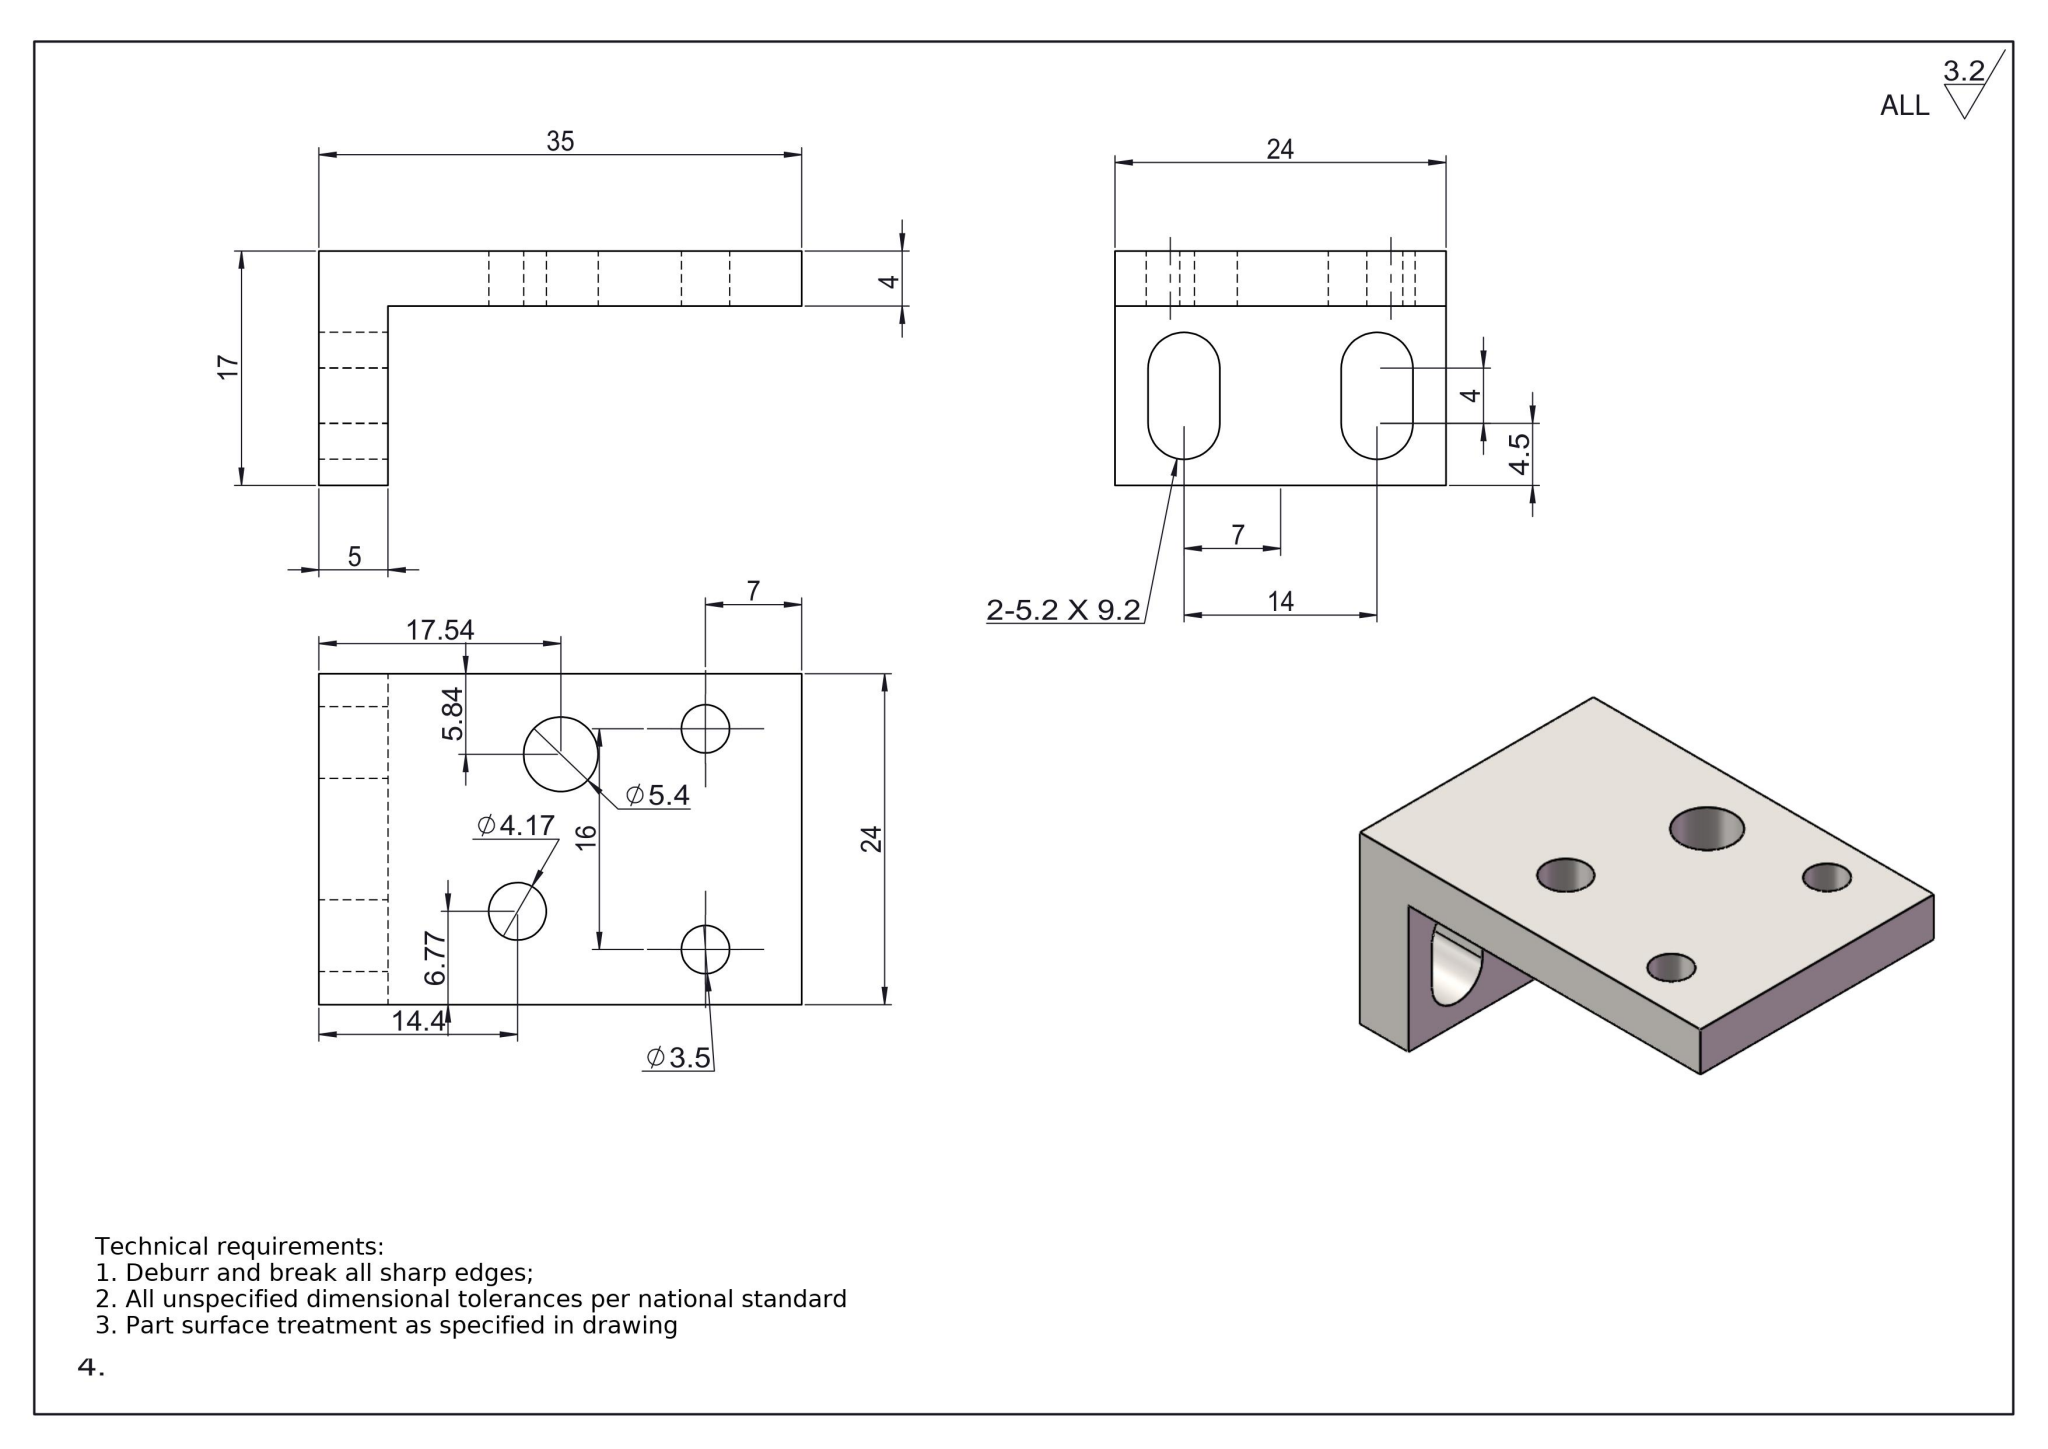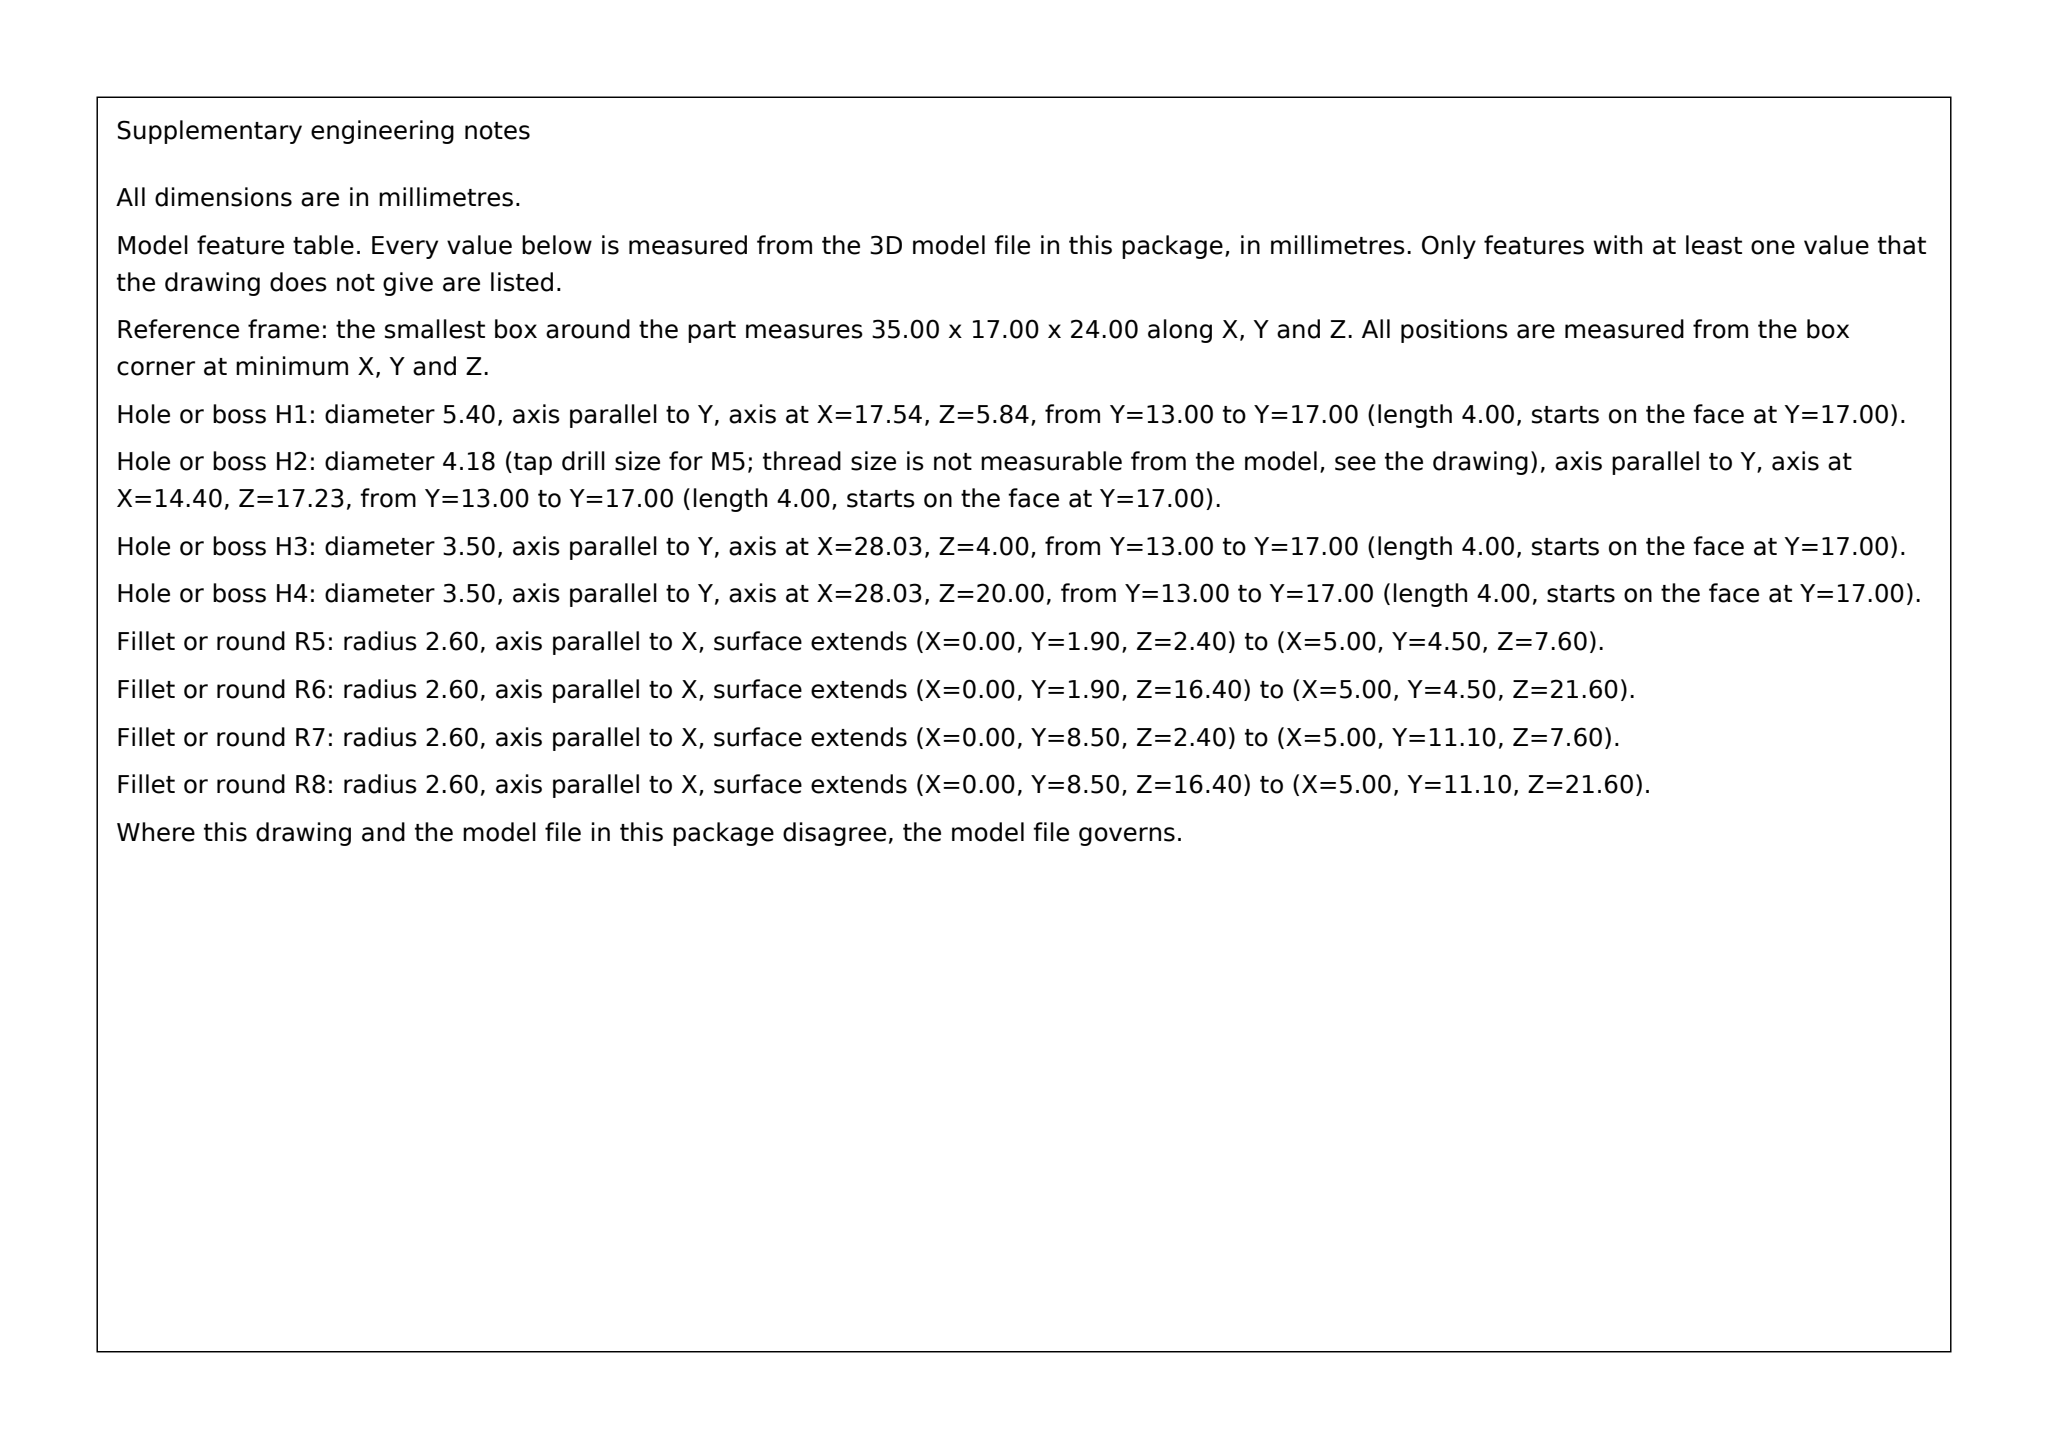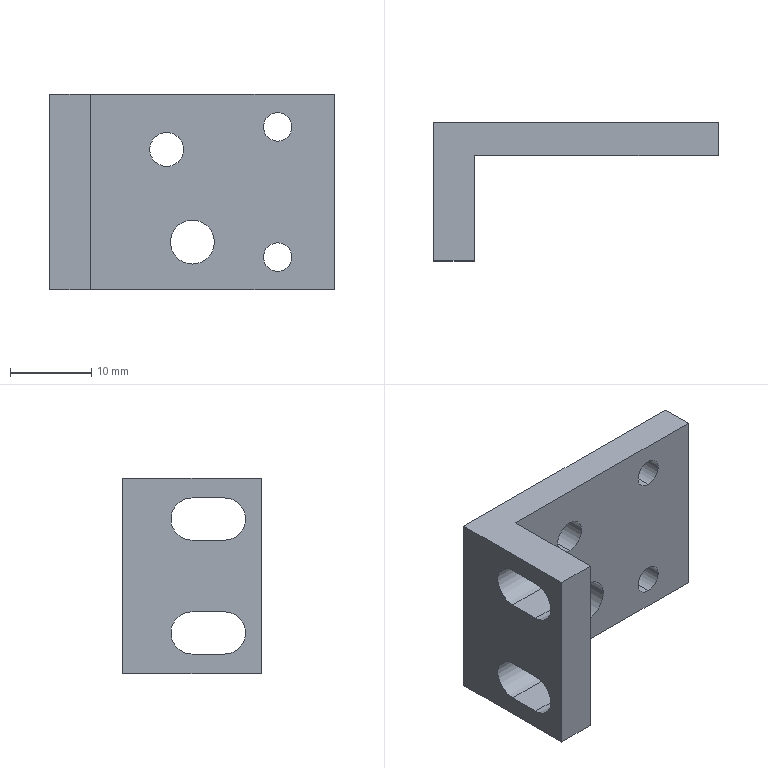Part | SolidWorks | mm | 1 solid | 24 faces | box 35 x 17 x 24 mm | volume 4276 mm3 | cylinder 12 | plane 12 | commonest cylinder face diameters 3.5 x4 5.2 x4 4.172 x2 5.404 x2
build123d program:
from build123d import *

# Parameters (mm, degrees)
BOSS_EXTRUDE1_DEPTH = 24
SKETCH2_R           = 1.75
CUT_EXTRUDE1_DEPTH  = 60.639
CUT_EXTRUDE2_DEPTH  = 46.946
SKETCH4_R           = 2.086
SKETCH4_R_2         = 2.702
CUT_EXTRUDE3_DEPTH  = 80


with BuildPart() as part:
    # Sketch1 → Boss-Extrude1 (new body)
    with BuildSketch(Plane.XY):
        Polygon((-53.027, -8.2), (-53.027, -25.2), (-48.027, -25.2), (-48.027, -12.2), (-18.027, -12.2), (-18.027, -8.2), align=None)
    extrude(amount=-BOSS_EXTRUDE1_DEPTH)

    # Sketch2 → Cut-Extrude1 (cut, through all)
    with BuildSketch(Plane.XZ.offset(12.2)):
        with Locations(Location((-25, -20, 0), (0, 0, 270))):
            Circle(SKETCH2_R)
        with Locations(Location((-25, -4, 0), (0, 0, 270))):
            Circle(SKETCH2_R)
    extrude(amount=-CUT_EXTRUDE1_DEPTH, mode=Mode.SUBTRACT)

    # Sketch3 → Cut-Extrude2 (cut, through all)
    with BuildSketch(Plane(origin=(-48.027, 0, 0), x_dir=(0, 0, -1), z_dir=(1, 0, 0))):
        with BuildLine():
            Line((7.6, -16.7), (7.6, -20.7))
            ThreePointArc((7.6, -20.7), (5, -23.3), (2.4, -20.7))
            Line((2.4, -20.7), (2.4, -16.7))
            ThreePointArc((2.4, -16.7), (5, -14.1), (7.6, -16.7))
        make_face()
        with BuildLine():
            Line((21.6, -16.7), (21.6, -20.7))
            ThreePointArc((21.6, -20.7), (19, -23.3), (16.4, -20.7))
            Line((16.4, -20.7), (16.4, -16.7))
            ThreePointArc((16.4, -16.7), (19, -14.1), (21.6, -16.7))
        make_face()
    extrude(amount=-CUT_EXTRUDE2_DEPTH, mode=Mode.SUBTRACT)

    # Sketch4 → Cut-Extrude3 (cut)
    with BuildSketch(Plane.XZ.offset(12.2)):
        with Locations(Location((-38.629, -6.772, 0), (0, 0, 270))):
            Circle(SKETCH4_R)
        with Locations(Location((-35.486, -18.158, 0), (0, 0, 270))):
            Circle(SKETCH4_R_2)
    extrude(amount=-CUT_EXTRUDE3_DEPTH, mode=Mode.SUBTRACT)


solid = part.part
STEP:
#1=CARTESIAN_POINT('',(-38.629,-8.2,-8.857));
#2=VERTEX_POINT('',#1);
#3=CARTESIAN_POINT('',(-38.629,-8.2,-4.686));
#4=VERTEX_POINT('',#3);
#5=CARTESIAN_POINT('',(-38.629,-8.2,-6.772));
#6=DIRECTION('',(0.,1.,0.));
#7=DIRECTION('',(-1.,0.,0.));
#8=AXIS2_PLACEMENT_3D('',#5,#6,#7);
#9=CIRCLE('',#8,2.086);
#10=EDGE_CURVE('',#2,#4,#9,.T.);
#11=ORIENTED_EDGE('',*,*,#10,.T.);
#12=CARTESIAN_POINT('',(-38.629,-12.2,-4.686));
#13=VERTEX_POINT('',#12);
#14=CARTESIAN_POINT('',(-38.629,67.8,-4.686));
#15=DIRECTION('',(0.,-1.,0.));
#16=VECTOR('',#15,1000.);
#17=LINE('',#14,#16);
#18=EDGE_CURVE('',#4,#13,#17,.T.);
#19=ORIENTED_EDGE('',*,*,#18,.T.);
#20=CARTESIAN_POINT('',(-38.629,-12.2,-8.857));
#21=VERTEX_POINT('',#20);
#22=CARTESIAN_POINT('',(-38.629,-12.2,-6.772));
#23=DIRECTION('',(0.,-1.,0.));
#24=DIRECTION('',(0.,0.,-1.));
#25=AXIS2_PLACEMENT_3D('',#22,#23,#24);
#26=CIRCLE('',#25,2.086);
#27=EDGE_CURVE('',#13,#21,#26,.T.);
#28=ORIENTED_EDGE('',*,*,#27,.T.);
#29=CARTESIAN_POINT('',(-38.629,67.8,-8.857));
#30=DIRECTION('',(0.,-1.,0.));
#31=VECTOR('',#30,1000.);
#32=LINE('',#29,#31);
#33=EDGE_CURVE('',#2,#21,#32,.T.);
#34=ORIENTED_EDGE('',*,*,#33,.F.);
#35=EDGE_LOOP('',(#11,#19,#28,#34));
#36=FACE_OUTER_BOUND('',#35,.T.);
#37=CARTESIAN_POINT('',(-38.629,67.8,-6.772));
#38=DIRECTION('',(0.,-1.,0.));
#39=DIRECTION('',(0.,0.,-1.));
#40=AXIS2_PLACEMENT_3D('',#37,#38,#39);
#41=CYLINDRICAL_SURFACE('',#40,2.086);
#42=ADVANCED_FACE('',(#36),#41,.F.);
#43=CARTESIAN_POINT('',(-35.486,-8.2,-20.86));
#44=VERTEX_POINT('',#43);
#45=CARTESIAN_POINT('',(-35.486,-8.2,-15.456));
#46=VERTEX_POINT('',#45);
#47=CARTESIAN_POINT('',(-35.486,-8.2,-18.158));
#48=DIRECTION('',(0.,1.,0.));
#49=DIRECTION('',(-1.,0.,0.));
#50=AXIS2_PLACEMENT_3D('',#47,#48,#49);
#51=CIRCLE('',#50,2.702);
#52=EDGE_CURVE('',#44,#46,#51,.T.);
#53=ORIENTED_EDGE('',*,*,#52,.T.);
#54=CARTESIAN_POINT('',(-35.486,-12.2,-15.456));
#55=VERTEX_POINT('',#54);
#56=CARTESIAN_POINT('',(-35.486,67.8,-15.456));
#57=DIRECTION('',(0.,-1.,0.));
#58=VECTOR('',#57,1000.);
#59=LINE('',#56,#58);
#60=EDGE_CURVE('',#46,#55,#59,.T.);
#61=ORIENTED_EDGE('',*,*,#60,.T.);
#62=CARTESIAN_POINT('',(-35.486,-12.2,-20.86));
#63=VERTEX_POINT('',#62);
#64=CARTESIAN_POINT('',(-35.486,-12.2,-18.158));
#65=DIRECTION('',(0.,-1.,0.));
#66=DIRECTION('',(0.,0.,-1.));
#67=AXIS2_PLACEMENT_3D('',#64,#65,#66);
#68=CIRCLE('',#67,2.702);
#69=EDGE_CURVE('',#55,#63,#68,.T.);
#70=ORIENTED_EDGE('',*,*,#69,.T.);
#71=CARTESIAN_POINT('',(-35.486,67.8,-20.86));
#72=DIRECTION('',(0.,-1.,0.));
#73=VECTOR('',#72,1000.);
#74=LINE('',#71,#73);
#75=EDGE_CURVE('',#44,#63,#74,.T.);
#76=ORIENTED_EDGE('',*,*,#75,.F.);
#77=EDGE_LOOP('',(#53,#61,#70,#76));
#78=FACE_OUTER_BOUND('',#77,.T.);
#79=CARTESIAN_POINT('',(-35.486,67.8,-18.158));
#80=DIRECTION('',(0.,-1.,0.));
#81=DIRECTION('',(0.,0.,-1.));
#82=AXIS2_PLACEMENT_3D('',#79,#80,#81);
#83=CYLINDRICAL_SURFACE('',#82,2.702);
#84=ADVANCED_FACE('',(#78),#83,.F.);
#85=CARTESIAN_POINT('',(-25.,-8.2,-2.25));
#86=VERTEX_POINT('',#85);
#87=CARTESIAN_POINT('',(-25.,-8.2,-5.75));
#88=VERTEX_POINT('',#87);
#89=CARTESIAN_POINT('',(-25.,-8.2,-4.));
#90=DIRECTION('',(0.,-1.,0.));
#91=DIRECTION('',(0.,0.,-1.));
#92=AXIS2_PLACEMENT_3D('',#89,#90,#91);
#93=CIRCLE('',#92,1.75);
#94=EDGE_CURVE('',#86,#88,#93,.T.);
#95=ORIENTED_EDGE('',*,*,#94,.F.);
#96=CARTESIAN_POINT('',(-25.,-12.2,-2.25));
#97=VERTEX_POINT('',#96);
#98=CARTESIAN_POINT('',(-25.,-8.2,-2.25));
#99=DIRECTION('',(0.,-1.,0.));
#100=VECTOR('',#99,1000.);
#101=LINE('',#98,#100);
#102=EDGE_CURVE('',#86,#97,#101,.T.);
#103=ORIENTED_EDGE('',*,*,#102,.T.);
#104=CARTESIAN_POINT('',(-25.,-12.2,-5.75));
#105=VERTEX_POINT('',#104);
#106=CARTESIAN_POINT('',(-25.,-12.2,-4.));
#107=DIRECTION('',(0.,-1.,0.));
#108=DIRECTION('',(0.,0.,-1.));
#109=AXIS2_PLACEMENT_3D('',#106,#107,#108);
#110=CIRCLE('',#109,1.75);
#111=EDGE_CURVE('',#97,#105,#110,.T.);
#112=ORIENTED_EDGE('',*,*,#111,.T.);
#113=CARTESIAN_POINT('',(-25.,-8.2,-5.75));
#114=DIRECTION('',(0.,-1.,0.));
#115=VECTOR('',#114,1000.);
#116=LINE('',#113,#115);
#117=EDGE_CURVE('',#88,#105,#116,.T.);
#118=ORIENTED_EDGE('',*,*,#117,.F.);
#119=EDGE_LOOP('',(#95,#103,#112,#118));
#120=FACE_OUTER_BOUND('',#119,.T.);
#121=CARTESIAN_POINT('',(-25.,-8.2,-4.));
#122=DIRECTION('',(0.,-1.,0.));
#123=DIRECTION('',(0.,0.,-1.));
#124=AXIS2_PLACEMENT_3D('',#121,#122,#123);
#125=CYLINDRICAL_SURFACE('',#124,1.75);
#126=ADVANCED_FACE('',(#120),#125,.F.);
#127=CARTESIAN_POINT('',(-25.,-8.2,-18.25));
#128=VERTEX_POINT('',#127);
#129=CARTESIAN_POINT('',(-25.,-8.2,-21.75));
#130=VERTEX_POINT('',#129);
#131=CARTESIAN_POINT('',(-25.,-8.2,-20.));
#132=DIRECTION('',(0.,-1.,0.));
#133=DIRECTION('',(0.,0.,-1.));
#134=AXIS2_PLACEMENT_3D('',#131,#132,#133);
#135=CIRCLE('',#134,1.75);
#136=EDGE_CURVE('',#128,#130,#135,.T.);
#137=ORIENTED_EDGE('',*,*,#136,.F.);
#138=CARTESIAN_POINT('',(-25.,-12.2,-18.25));
#139=VERTEX_POINT('',#138);
#140=CARTESIAN_POINT('',(-25.,-8.2,-18.25));
#141=DIRECTION('',(0.,-1.,0.));
#142=VECTOR('',#141,1000.);
#143=LINE('',#140,#142);
#144=EDGE_CURVE('',#128,#139,#143,.T.);
#145=ORIENTED_EDGE('',*,*,#144,.T.);
#146=CARTESIAN_POINT('',(-25.,-12.2,-21.75));
#147=VERTEX_POINT('',#146);
#148=CARTESIAN_POINT('',(-25.,-12.2,-20.));
#149=DIRECTION('',(0.,-1.,0.));
#150=DIRECTION('',(0.,0.,-1.));
#151=AXIS2_PLACEMENT_3D('',#148,#149,#150);
#152=CIRCLE('',#151,1.75);
#153=EDGE_CURVE('',#139,#147,#152,.T.);
#154=ORIENTED_EDGE('',*,*,#153,.T.);
#155=CARTESIAN_POINT('',(-25.,-8.2,-21.75));
#156=DIRECTION('',(0.,-1.,0.));
#157=VECTOR('',#156,1000.);
#158=LINE('',#155,#157);
#159=EDGE_CURVE('',#130,#147,#158,.T.);
#160=ORIENTED_EDGE('',*,*,#159,.F.);
#161=EDGE_LOOP('',(#137,#145,#154,#160));
#162=FACE_OUTER_BOUND('',#161,.T.);
#163=CARTESIAN_POINT('',(-25.,-8.2,-20.));
#164=DIRECTION('',(0.,-1.,0.));
#165=DIRECTION('',(0.,0.,-1.));
#166=AXIS2_PLACEMENT_3D('',#163,#164,#165);
#167=CYLINDRICAL_SURFACE('',#166,1.75);
#168=ADVANCED_FACE('',(#162),#167,.F.);
#169=ORIENTED_EDGE('',*,*,#10,.F.);
#170=CARTESIAN_POINT('',(-38.629,-8.2,-6.772));
#171=DIRECTION('',(0.,1.,0.));
#172=DIRECTION('',(-1.,0.,0.));
#173=AXIS2_PLACEMENT_3D('',#170,#171,#172);
#174=CIRCLE('',#173,2.086);
#175=EDGE_CURVE('',#4,#2,#174,.T.);
#176=ORIENTED_EDGE('',*,*,#175,.F.);
#177=EDGE_LOOP('',(#169,#176));
#178=FACE_BOUND('',#177,.T.);
#179=ORIENTED_EDGE('',*,*,#52,.F.);
#180=CARTESIAN_POINT('',(-35.486,-8.2,-18.158));
#181=DIRECTION('',(0.,1.,0.));
#182=DIRECTION('',(-1.,0.,0.));
#183=AXIS2_PLACEMENT_3D('',#180,#181,#182);
#184=CIRCLE('',#183,2.702);
#185=EDGE_CURVE('',#46,#44,#184,.T.);
#186=ORIENTED_EDGE('',*,*,#185,.F.);
#187=EDGE_LOOP('',(#179,#186));
#188=FACE_BOUND('',#187,.T.);
#189=CARTESIAN_POINT('',(-25.,-8.2,-4.));
#190=DIRECTION('',(0.,-1.,0.));
#191=DIRECTION('',(0.,0.,-1.));
#192=AXIS2_PLACEMENT_3D('',#189,#190,#191);
#193=CIRCLE('',#192,1.75);
#194=EDGE_CURVE('',#88,#86,#193,.T.);
#195=ORIENTED_EDGE('',*,*,#194,.T.);
#196=ORIENTED_EDGE('',*,*,#94,.T.);
#197=EDGE_LOOP('',(#195,#196));
#198=FACE_BOUND('',#197,.T.);
#199=CARTESIAN_POINT('',(-25.,-8.2,-20.));
#200=DIRECTION('',(0.,-1.,0.));
#201=DIRECTION('',(0.,0.,-1.));
#202=AXIS2_PLACEMENT_3D('',#199,#200,#201);
#203=CIRCLE('',#202,1.75);
#204=EDGE_CURVE('',#130,#128,#203,.T.);
#205=ORIENTED_EDGE('',*,*,#204,.T.);
#206=ORIENTED_EDGE('',*,*,#136,.T.);
#207=EDGE_LOOP('',(#205,#206));
#208=FACE_BOUND('',#207,.T.);
#209=CARTESIAN_POINT('',(-18.027,-8.2,0.));
#210=VERTEX_POINT('',#209);
#211=CARTESIAN_POINT('',(-53.027,-8.2,0.));
#212=VERTEX_POINT('',#211);
#213=CARTESIAN_POINT('',(-18.027,-8.2,0.));
#214=DIRECTION('',(-1.,0.,0.));
#215=VECTOR('',#214,1000.);
#216=LINE('',#213,#215);
#217=EDGE_CURVE('',#210,#212,#216,.T.);
#218=ORIENTED_EDGE('',*,*,#217,.F.);
#219=CARTESIAN_POINT('',(-18.027,-8.2,-24.));
#220=VERTEX_POINT('',#219);
#221=CARTESIAN_POINT('',(-18.027,-8.2,-24.));
#222=DIRECTION('',(0.,0.,1.));
#223=VECTOR('',#222,1000.);
#224=LINE('',#221,#223);
#225=EDGE_CURVE('',#220,#210,#224,.T.);
#226=ORIENTED_EDGE('',*,*,#225,.F.);
#227=CARTESIAN_POINT('',(-53.027,-8.2,-24.));
#228=VERTEX_POINT('',#227);
#229=CARTESIAN_POINT('',(-18.027,-8.2,-24.));
#230=DIRECTION('',(-1.,0.,0.));
#231=VECTOR('',#230,1000.);
#232=LINE('',#229,#231);
#233=EDGE_CURVE('',#220,#228,#232,.T.);
#234=ORIENTED_EDGE('',*,*,#233,.T.);
#235=CARTESIAN_POINT('',(-53.027,-8.2,-24.));
#236=DIRECTION('',(0.,0.,1.));
#237=VECTOR('',#236,1000.);
#238=LINE('',#235,#237);
#239=EDGE_CURVE('',#228,#212,#238,.T.);
#240=ORIENTED_EDGE('',*,*,#239,.T.);
#241=EDGE_LOOP('',(#218,#226,#234,#240));
#242=FACE_OUTER_BOUND('',#241,.T.);
#243=CARTESIAN_POINT('',(-18.027,-8.2,-24.));
#244=DIRECTION('',(0.,1.,0.));
#245=DIRECTION('',(-1.,0.,0.));
#246=AXIS2_PLACEMENT_3D('',#243,#244,#245);
#247=PLANE('',#246);
#248=ADVANCED_FACE('',(#178,#188,#198,#208,#242),#247,.T.);
#249=CARTESIAN_POINT('',(-18.027,-12.2,0.));
#250=VERTEX_POINT('',#249);
#251=CARTESIAN_POINT('',(-18.027,-12.2,0.));
#252=DIRECTION('',(0.,1.,0.));
#253=VECTOR('',#252,1000.);
#254=LINE('',#251,#253);
#255=EDGE_CURVE('',#250,#210,#254,.T.);
#256=ORIENTED_EDGE('',*,*,#255,.F.);
#257=CARTESIAN_POINT('',(-18.027,-12.2,-24.));
#258=VERTEX_POINT('',#257);
#259=CARTESIAN_POINT('',(-18.027,-12.2,-24.));
#260=DIRECTION('',(0.,0.,1.));
#261=VECTOR('',#260,1000.);
#262=LINE('',#259,#261);
#263=EDGE_CURVE('',#258,#250,#262,.T.);
#264=ORIENTED_EDGE('',*,*,#263,.F.);
#265=CARTESIAN_POINT('',(-18.027,-12.2,-24.));
#266=DIRECTION('',(0.,1.,0.));
#267=VECTOR('',#266,1000.);
#268=LINE('',#265,#267);
#269=EDGE_CURVE('',#258,#220,#268,.T.);
#270=ORIENTED_EDGE('',*,*,#269,.T.);
#271=ORIENTED_EDGE('',*,*,#225,.T.);
#272=EDGE_LOOP('',(#256,#264,#270,#271));
#273=FACE_OUTER_BOUND('',#272,.T.);
#274=CARTESIAN_POINT('',(-18.027,-12.2,-24.));
#275=DIRECTION('',(1.,0.,0.));
#276=DIRECTION('',(0.,0.,-1.));
#277=AXIS2_PLACEMENT_3D('',#274,#275,#276);
#278=PLANE('',#277);
#279=ADVANCED_FACE('',(#273),#278,.T.);
#280=CARTESIAN_POINT('',(-38.629,-12.2,-6.772));
#281=DIRECTION('',(0.,-1.,0.));
#282=DIRECTION('',(0.,0.,-1.));
#283=AXIS2_PLACEMENT_3D('',#280,#281,#282);
#284=CIRCLE('',#283,2.086);
#285=EDGE_CURVE('',#21,#13,#284,.T.);
#286=ORIENTED_EDGE('',*,*,#285,.F.);
#287=ORIENTED_EDGE('',*,*,#27,.F.);
#288=EDGE_LOOP('',(#286,#287));
#289=FACE_BOUND('',#288,.T.);
#290=CARTESIAN_POINT('',(-35.486,-12.2,-18.158));
#291=DIRECTION('',(0.,-1.,0.));
#292=DIRECTION('',(0.,0.,-1.));
#293=AXIS2_PLACEMENT_3D('',#290,#291,#292);
#294=CIRCLE('',#293,2.702);
#295=EDGE_CURVE('',#63,#55,#294,.T.);
#296=ORIENTED_EDGE('',*,*,#295,.F.);
#297=ORIENTED_EDGE('',*,*,#69,.F.);
#298=EDGE_LOOP('',(#296,#297));
#299=FACE_BOUND('',#298,.T.);
#300=CARTESIAN_POINT('',(-25.,-12.2,-4.));
#301=DIRECTION('',(0.,-1.,0.));
#302=DIRECTION('',(0.,0.,-1.));
#303=AXIS2_PLACEMENT_3D('',#300,#301,#302);
#304=CIRCLE('',#303,1.75);
#305=EDGE_CURVE('',#105,#97,#304,.T.);
#306=ORIENTED_EDGE('',*,*,#305,.F.);
#307=ORIENTED_EDGE('',*,*,#111,.F.);
#308=EDGE_LOOP('',(#306,#307));
#309=FACE_BOUND('',#308,.T.);
#310=CARTESIAN_POINT('',(-25.,-12.2,-20.));
#311=DIRECTION('',(0.,-1.,0.));
#312=DIRECTION('',(0.,0.,-1.));
#313=AXIS2_PLACEMENT_3D('',#310,#311,#312);
#314=CIRCLE('',#313,1.75);
#315=EDGE_CURVE('',#147,#139,#314,.T.);
#316=ORIENTED_EDGE('',*,*,#315,.F.);
#317=ORIENTED_EDGE('',*,*,#153,.F.);
#318=EDGE_LOOP('',(#316,#317));
#319=FACE_BOUND('',#318,.T.);
#320=CARTESIAN_POINT('',(-48.027,-12.2,0.));
#321=VERTEX_POINT('',#320);
#322=CARTESIAN_POINT('',(-48.027,-12.2,0.));
#323=DIRECTION('',(1.,0.,0.));
#324=VECTOR('',#323,1000.);
#325=LINE('',#322,#324);
#326=EDGE_CURVE('',#321,#250,#325,.T.);
#327=ORIENTED_EDGE('',*,*,#326,.F.);
#328=CARTESIAN_POINT('',(-48.027,-12.2,-24.));
#329=VERTEX_POINT('',#328);
#330=CARTESIAN_POINT('',(-48.027,-12.2,-24.));
#331=DIRECTION('',(0.,0.,1.));
#332=VECTOR('',#331,1000.);
#333=LINE('',#330,#332);
#334=EDGE_CURVE('',#329,#321,#333,.T.);
#335=ORIENTED_EDGE('',*,*,#334,.F.);
#336=CARTESIAN_POINT('',(-48.027,-12.2,-24.));
#337=DIRECTION('',(1.,0.,0.));
#338=VECTOR('',#337,1000.);
#339=LINE('',#336,#338);
#340=EDGE_CURVE('',#329,#258,#339,.T.);
#341=ORIENTED_EDGE('',*,*,#340,.T.);
#342=ORIENTED_EDGE('',*,*,#263,.T.);
#343=EDGE_LOOP('',(#327,#335,#341,#342));
#344=FACE_OUTER_BOUND('',#343,.T.);
#345=CARTESIAN_POINT('',(-48.027,-12.2,-24.));
#346=DIRECTION('',(0.,-1.,0.));
#347=DIRECTION('',(0.,0.,-1.));
#348=AXIS2_PLACEMENT_3D('',#345,#346,#347);
#349=PLANE('',#348);
#350=ADVANCED_FACE('',(#289,#299,#309,#319,#344),#349,.T.);
#351=CARTESIAN_POINT('',(-48.027,-16.7,-21.6));
#352=VERTEX_POINT('',#351);
#353=CARTESIAN_POINT('',(-48.027,-16.7,-16.4));
#354=VERTEX_POINT('',#353);
#355=CARTESIAN_POINT('',(-48.027,-16.7,-19.));
#356=DIRECTION('',(1.,0.,0.));
#357=DIRECTION('',(0.,0.,-1.));
#358=AXIS2_PLACEMENT_3D('',#355,#356,#357);
#359=CIRCLE('',#358,2.6);
#360=EDGE_CURVE('',#352,#354,#359,.T.);
#361=ORIENTED_EDGE('',*,*,#360,.F.);
#362=CARTESIAN_POINT('',(-48.027,-20.7,-21.6));
#363=VERTEX_POINT('',#362);
#364=CARTESIAN_POINT('',(-48.027,-16.7,-21.6));
#365=DIRECTION('',(0.,1.,0.));
#366=VECTOR('',#365,1000.);
#367=LINE('',#364,#366);
#368=EDGE_CURVE('',#363,#352,#367,.T.);
#369=ORIENTED_EDGE('',*,*,#368,.F.);
#370=CARTESIAN_POINT('',(-48.027,-20.7,-16.4));
#371=VERTEX_POINT('',#370);
#372=CARTESIAN_POINT('',(-48.027,-20.7,-19.));
#373=DIRECTION('',(1.,0.,0.));
#374=DIRECTION('',(0.,0.,-1.));
#375=AXIS2_PLACEMENT_3D('',#372,#373,#374);
#376=CIRCLE('',#375,2.6);
#377=EDGE_CURVE('',#371,#363,#376,.T.);
#378=ORIENTED_EDGE('',*,*,#377,.F.);
#379=CARTESIAN_POINT('',(-48.027,-16.7,-16.4));
#380=DIRECTION('',(0.,-1.,0.));
#381=VECTOR('',#380,1000.);
#382=LINE('',#379,#381);
#383=EDGE_CURVE('',#354,#371,#382,.T.);
#384=ORIENTED_EDGE('',*,*,#383,.F.);
#385=EDGE_LOOP('',(#361,#369,#378,#384));
#386=FACE_BOUND('',#385,.T.);
#387=CARTESIAN_POINT('',(-48.027,-16.7,-7.6));
#388=VERTEX_POINT('',#387);
#389=CARTESIAN_POINT('',(-48.027,-16.7,-2.4));
#390=VERTEX_POINT('',#389);
#391=CARTESIAN_POINT('',(-48.027,-16.7,-5.));
#392=DIRECTION('',(1.,0.,0.));
#393=DIRECTION('',(0.,0.,-1.));
#394=AXIS2_PLACEMENT_3D('',#391,#392,#393);
#395=CIRCLE('',#394,2.6);
#396=EDGE_CURVE('',#388,#390,#395,.T.);
#397=ORIENTED_EDGE('',*,*,#396,.F.);
#398=CARTESIAN_POINT('',(-48.027,-20.7,-7.6));
#399=VERTEX_POINT('',#398);
#400=CARTESIAN_POINT('',(-48.027,-16.7,-7.6));
#401=DIRECTION('',(0.,1.,0.));
#402=VECTOR('',#401,1000.);
#403=LINE('',#400,#402);
#404=EDGE_CURVE('',#399,#388,#403,.T.);
#405=ORIENTED_EDGE('',*,*,#404,.F.);
#406=CARTESIAN_POINT('',(-48.027,-20.7,-2.4));
#407=VERTEX_POINT('',#406);
#408=CARTESIAN_POINT('',(-48.027,-20.7,-5.));
#409=DIRECTION('',(1.,0.,0.));
#410=DIRECTION('',(0.,0.,-1.));
#411=AXIS2_PLACEMENT_3D('',#408,#409,#410);
#412=CIRCLE('',#411,2.6);
#413=EDGE_CURVE('',#407,#399,#412,.T.);
#414=ORIENTED_EDGE('',*,*,#413,.F.);
#415=CARTESIAN_POINT('',(-48.027,-16.7,-2.4));
#416=DIRECTION('',(0.,-1.,-0.));
#417=VECTOR('',#416,1000.);
#418=LINE('',#415,#417);
#419=EDGE_CURVE('',#390,#407,#418,.T.);
#420=ORIENTED_EDGE('',*,*,#419,.F.);
#421=EDGE_LOOP('',(#397,#405,#414,#420));
#422=FACE_BOUND('',#421,.T.);
#423=CARTESIAN_POINT('',(-48.027,-25.2,0.));
#424=VERTEX_POINT('',#423);
#425=CARTESIAN_POINT('',(-48.027,-25.2,0.));
#426=DIRECTION('',(0.,1.,0.));
#427=VECTOR('',#426,1000.);
#428=LINE('',#425,#427);
#429=EDGE_CURVE('',#424,#321,#428,.T.);
#430=ORIENTED_EDGE('',*,*,#429,.F.);
#431=CARTESIAN_POINT('',(-48.027,-25.2,-24.));
#432=VERTEX_POINT('',#431);
#433=CARTESIAN_POINT('',(-48.027,-25.2,-24.));
#434=DIRECTION('',(0.,0.,1.));
#435=VECTOR('',#434,1000.);
#436=LINE('',#433,#435);
#437=EDGE_CURVE('',#432,#424,#436,.T.);
#438=ORIENTED_EDGE('',*,*,#437,.F.);
#439=CARTESIAN_POINT('',(-48.027,-25.2,-24.));
#440=DIRECTION('',(0.,1.,0.));
#441=VECTOR('',#440,1000.);
#442=LINE('',#439,#441);
#443=EDGE_CURVE('',#432,#329,#442,.T.);
#444=ORIENTED_EDGE('',*,*,#443,.T.);
#445=ORIENTED_EDGE('',*,*,#334,.T.);
#446=EDGE_LOOP('',(#430,#438,#444,#445));
#447=FACE_OUTER_BOUND('',#446,.T.);
#448=CARTESIAN_POINT('',(-48.027,-25.2,-24.));
#449=DIRECTION('',(1.,0.,0.));
#450=DIRECTION('',(0.,0.,-1.));
#451=AXIS2_PLACEMENT_3D('',#448,#449,#450);
#452=PLANE('',#451);
#453=ADVANCED_FACE('',(#386,#422,#447),#452,.T.);
#454=CARTESIAN_POINT('',(-53.027,-25.2,0.));
#455=VERTEX_POINT('',#454);
#456=CARTESIAN_POINT('',(-53.027,-25.2,0.));
#457=DIRECTION('',(1.,0.,0.));
#458=VECTOR('',#457,1000.);
#459=LINE('',#456,#458);
#460=EDGE_CURVE('',#455,#424,#459,.T.);
#461=ORIENTED_EDGE('',*,*,#460,.F.);
#462=CARTESIAN_POINT('',(-53.027,-25.2,-24.));
#463=VERTEX_POINT('',#462);
#464=CARTESIAN_POINT('',(-53.027,-25.2,-24.));
#465=DIRECTION('',(0.,0.,1.));
#466=VECTOR('',#465,1000.);
#467=LINE('',#464,#466);
#468=EDGE_CURVE('',#463,#455,#467,.T.);
#469=ORIENTED_EDGE('',*,*,#468,.F.);
#470=CARTESIAN_POINT('',(-53.027,-25.2,-24.));
#471=DIRECTION('',(1.,0.,0.));
#472=VECTOR('',#471,1000.);
#473=LINE('',#470,#472);
#474=EDGE_CURVE('',#463,#432,#473,.T.);
#475=ORIENTED_EDGE('',*,*,#474,.T.);
#476=ORIENTED_EDGE('',*,*,#437,.T.);
#477=EDGE_LOOP('',(#461,#469,#475,#476));
#478=FACE_OUTER_BOUND('',#477,.T.);
#479=CARTESIAN_POINT('',(-53.027,-25.2,-24.));
#480=DIRECTION('',(0.,-1.,0.));
#481=DIRECTION('',(0.,0.,-1.));
#482=AXIS2_PLACEMENT_3D('',#479,#480,#481);
#483=PLANE('',#482);
#484=ADVANCED_FACE('',(#478),#483,.T.);
#485=CARTESIAN_POINT('',(-53.027,-16.7,-21.6));
#486=VERTEX_POINT('',#485);
#487=CARTESIAN_POINT('',(-53.027,-16.7,-16.4));
#488=VERTEX_POINT('',#487);
#489=CARTESIAN_POINT('',(-53.027,-16.7,-19.));
#490=DIRECTION('',(1.,0.,0.));
#491=DIRECTION('',(0.,0.,-1.));
#492=AXIS2_PLACEMENT_3D('',#489,#490,#491);
#493=CIRCLE('',#492,2.6);
#494=EDGE_CURVE('',#486,#488,#493,.T.);
#495=ORIENTED_EDGE('',*,*,#494,.T.);
#496=CARTESIAN_POINT('',(-53.027,-20.7,-16.4));
#497=VERTEX_POINT('',#496);
#498=CARTESIAN_POINT('',(-53.027,-16.7,-16.4));
#499=DIRECTION('',(0.,-1.,0.));
#500=VECTOR('',#499,1000.);
#501=LINE('',#498,#500);
#502=EDGE_CURVE('',#488,#497,#501,.T.);
#503=ORIENTED_EDGE('',*,*,#502,.T.);
#504=CARTESIAN_POINT('',(-53.027,-20.7,-21.6));
#505=VERTEX_POINT('',#504);
#506=CARTESIAN_POINT('',(-53.027,-20.7,-19.));
#507=DIRECTION('',(1.,0.,0.));
#508=DIRECTION('',(0.,0.,-1.));
#509=AXIS2_PLACEMENT_3D('',#506,#507,#508);
#510=CIRCLE('',#509,2.6);
#511=EDGE_CURVE('',#497,#505,#510,.T.);
#512=ORIENTED_EDGE('',*,*,#511,.T.);
#513=CARTESIAN_POINT('',(-53.027,-16.7,-21.6));
#514=DIRECTION('',(0.,1.,0.));
#515=VECTOR('',#514,1000.);
#516=LINE('',#513,#515);
#517=EDGE_CURVE('',#505,#486,#516,.T.);
#518=ORIENTED_EDGE('',*,*,#517,.T.);
#519=EDGE_LOOP('',(#495,#503,#512,#518));
#520=FACE_BOUND('',#519,.T.);
#521=CARTESIAN_POINT('',(-53.027,-16.7,-7.6));
#522=VERTEX_POINT('',#521);
#523=CARTESIAN_POINT('',(-53.027,-16.7,-2.4));
#524=VERTEX_POINT('',#523);
#525=CARTESIAN_POINT('',(-53.027,-16.7,-5.));
#526=DIRECTION('',(1.,0.,0.));
#527=DIRECTION('',(0.,0.,-1.));
#528=AXIS2_PLACEMENT_3D('',#525,#526,#527);
#529=CIRCLE('',#528,2.6);
#530=EDGE_CURVE('',#522,#524,#529,.T.);
#531=ORIENTED_EDGE('',*,*,#530,.T.);
#532=CARTESIAN_POINT('',(-53.027,-20.7,-2.4));
#533=VERTEX_POINT('',#532);
#534=CARTESIAN_POINT('',(-53.027,-16.7,-2.4));
#535=DIRECTION('',(0.,-1.,-0.));
#536=VECTOR('',#535,1000.);
#537=LINE('',#534,#536);
#538=EDGE_CURVE('',#524,#533,#537,.T.);
#539=ORIENTED_EDGE('',*,*,#538,.T.);
#540=CARTESIAN_POINT('',(-53.027,-20.7,-7.6));
#541=VERTEX_POINT('',#540);
#542=CARTESIAN_POINT('',(-53.027,-20.7,-5.));
#543=DIRECTION('',(1.,0.,0.));
#544=DIRECTION('',(0.,0.,-1.));
#545=AXIS2_PLACEMENT_3D('',#542,#543,#544);
#546=CIRCLE('',#545,2.6);
#547=EDGE_CURVE('',#533,#541,#546,.T.);
#548=ORIENTED_EDGE('',*,*,#547,.T.);
#549=CARTESIAN_POINT('',(-53.027,-16.7,-7.6));
#550=DIRECTION('',(0.,1.,0.));
#551=VECTOR('',#550,1000.);
#552=LINE('',#549,#551);
#553=EDGE_CURVE('',#541,#522,#552,.T.);
#554=ORIENTED_EDGE('',*,*,#553,.T.);
#555=EDGE_LOOP('',(#531,#539,#548,#554));
#556=FACE_BOUND('',#555,.T.);
#557=CARTESIAN_POINT('',(-53.027,-8.2,0.));
#558=DIRECTION('',(0.,-1.,0.));
#559=VECTOR('',#558,1000.);
#560=LINE('',#557,#559);
#561=EDGE_CURVE('',#212,#455,#560,.T.);
#562=ORIENTED_EDGE('',*,*,#561,.F.);
#563=ORIENTED_EDGE('',*,*,#239,.F.);
#564=CARTESIAN_POINT('',(-53.027,-8.2,-24.));
#565=DIRECTION('',(0.,-1.,0.));
#566=VECTOR('',#565,1000.);
#567=LINE('',#564,#566);
#568=EDGE_CURVE('',#228,#463,#567,.T.);
#569=ORIENTED_EDGE('',*,*,#568,.T.);
#570=ORIENTED_EDGE('',*,*,#468,.T.);
#571=EDGE_LOOP('',(#562,#563,#569,#570));
#572=FACE_OUTER_BOUND('',#571,.T.);
#573=CARTESIAN_POINT('',(-53.027,-8.2,-24.));
#574=DIRECTION('',(-1.,0.,0.));
#575=DIRECTION('',(0.,0.,1.));
#576=AXIS2_PLACEMENT_3D('',#573,#574,#575);
#577=PLANE('',#576);
#578=ADVANCED_FACE('',(#520,#556,#572),#577,.T.);
#579=ORIENTED_EDGE('',*,*,#233,.F.);
#580=ORIENTED_EDGE('',*,*,#269,.F.);
#581=ORIENTED_EDGE('',*,*,#340,.F.);
#582=ORIENTED_EDGE('',*,*,#443,.F.);
#583=ORIENTED_EDGE('',*,*,#474,.F.);
#584=ORIENTED_EDGE('',*,*,#568,.F.);
#585=EDGE_LOOP('',(#579,#580,#581,#582,#583,#584));
#586=FACE_OUTER_BOUND('',#585,.T.);
#587=CARTESIAN_POINT('',(0.,0.,-24.));
#588=DIRECTION('',(0.,0.,1.));
#589=DIRECTION('',(1.,0.,0.));
#590=AXIS2_PLACEMENT_3D('',#587,#588,#589);
#591=PLANE('',#590);
#592=ADVANCED_FACE('',(#586),#591,.F.);
#593=ORIENTED_EDGE('',*,*,#217,.T.);
#594=ORIENTED_EDGE('',*,*,#561,.T.);
#595=ORIENTED_EDGE('',*,*,#460,.T.);
#596=ORIENTED_EDGE('',*,*,#429,.T.);
#597=ORIENTED_EDGE('',*,*,#326,.T.);
#598=ORIENTED_EDGE('',*,*,#255,.T.);
#599=EDGE_LOOP('',(#593,#594,#595,#596,#597,#598));
#600=FACE_OUTER_BOUND('',#599,.T.);
#601=CARTESIAN_POINT('',(0.,0.,0.));
#602=DIRECTION('',(0.,0.,1.));
#603=DIRECTION('',(1.,0.,0.));
#604=AXIS2_PLACEMENT_3D('',#601,#602,#603);
#605=PLANE('',#604);
#606=ADVANCED_FACE('',(#600),#605,.T.);
#607=ORIENTED_EDGE('',*,*,#144,.F.);
#608=ORIENTED_EDGE('',*,*,#204,.F.);
#609=ORIENTED_EDGE('',*,*,#159,.T.);
#610=ORIENTED_EDGE('',*,*,#315,.T.);
#611=EDGE_LOOP('',(#607,#608,#609,#610));
#612=FACE_OUTER_BOUND('',#611,.T.);
#613=CARTESIAN_POINT('',(-25.,-8.2,-20.));
#614=DIRECTION('',(0.,-1.,0.));
#615=DIRECTION('',(0.,0.,-1.));
#616=AXIS2_PLACEMENT_3D('',#613,#614,#615);
#617=CYLINDRICAL_SURFACE('',#616,1.75);
#618=ADVANCED_FACE('',(#612),#617,.F.);
#619=ORIENTED_EDGE('',*,*,#102,.F.);
#620=ORIENTED_EDGE('',*,*,#194,.F.);
#621=ORIENTED_EDGE('',*,*,#117,.T.);
#622=ORIENTED_EDGE('',*,*,#305,.T.);
#623=EDGE_LOOP('',(#619,#620,#621,#622));
#624=FACE_OUTER_BOUND('',#623,.T.);
#625=CARTESIAN_POINT('',(-25.,-8.2,-4.));
#626=DIRECTION('',(0.,-1.,0.));
#627=DIRECTION('',(0.,0.,-1.));
#628=AXIS2_PLACEMENT_3D('',#625,#626,#627);
#629=CYLINDRICAL_SURFACE('',#628,1.75);
#630=ADVANCED_FACE('',(#624),#629,.F.);
#631=ORIENTED_EDGE('',*,*,#396,.T.);
#632=CARTESIAN_POINT('',(-53.027,-16.7,-2.4));
#633=DIRECTION('',(1.,0.,0.));
#634=VECTOR('',#633,1000.);
#635=LINE('',#632,#634);
#636=EDGE_CURVE('',#524,#390,#635,.T.);
#637=ORIENTED_EDGE('',*,*,#636,.F.);
#638=ORIENTED_EDGE('',*,*,#530,.F.);
#639=CARTESIAN_POINT('',(-53.027,-16.7,-7.6));
#640=DIRECTION('',(1.,0.,0.));
#641=VECTOR('',#640,1000.);
#642=LINE('',#639,#641);
#643=EDGE_CURVE('',#522,#388,#642,.T.);
#644=ORIENTED_EDGE('',*,*,#643,.T.);
#645=EDGE_LOOP('',(#631,#637,#638,#644));
#646=FACE_OUTER_BOUND('',#645,.T.);
#647=CARTESIAN_POINT('',(-53.027,-16.7,-5.));
#648=DIRECTION('',(1.,0.,0.));
#649=DIRECTION('',(0.,0.,-1.));
#650=AXIS2_PLACEMENT_3D('',#647,#648,#649);
#651=CYLINDRICAL_SURFACE('',#650,2.6);
#652=ADVANCED_FACE('',(#646),#651,.F.);
#653=ORIENTED_EDGE('',*,*,#404,.T.);
#654=ORIENTED_EDGE('',*,*,#643,.F.);
#655=ORIENTED_EDGE('',*,*,#553,.F.);
#656=CARTESIAN_POINT('',(-53.027,-20.7,-7.6));
#657=DIRECTION('',(1.,0.,0.));
#658=VECTOR('',#657,1000.);
#659=LINE('',#656,#658);
#660=EDGE_CURVE('',#541,#399,#659,.T.);
#661=ORIENTED_EDGE('',*,*,#660,.T.);
#662=EDGE_LOOP('',(#653,#654,#655,#661));
#663=FACE_OUTER_BOUND('',#662,.T.);
#664=CARTESIAN_POINT('',(-53.027,-16.7,-7.6));
#665=DIRECTION('',(0.,0.,-1.));
#666=DIRECTION('',(0.,1.,0.));
#667=AXIS2_PLACEMENT_3D('',#664,#665,#666);
#668=PLANE('',#667);
#669=ADVANCED_FACE('',(#663),#668,.F.);
#670=ORIENTED_EDGE('',*,*,#413,.T.);
#671=ORIENTED_EDGE('',*,*,#660,.F.);
#672=ORIENTED_EDGE('',*,*,#547,.F.);
#673=CARTESIAN_POINT('',(-53.027,-20.7,-2.4));
#674=DIRECTION('',(1.,0.,0.));
#675=VECTOR('',#674,1000.);
#676=LINE('',#673,#675);
#677=EDGE_CURVE('',#533,#407,#676,.T.);
#678=ORIENTED_EDGE('',*,*,#677,.T.);
#679=EDGE_LOOP('',(#670,#671,#672,#678));
#680=FACE_OUTER_BOUND('',#679,.T.);
#681=CARTESIAN_POINT('',(-53.027,-20.7,-5.));
#682=DIRECTION('',(1.,0.,0.));
#683=DIRECTION('',(0.,0.,-1.));
#684=AXIS2_PLACEMENT_3D('',#681,#682,#683);
#685=CYLINDRICAL_SURFACE('',#684,2.6);
#686=ADVANCED_FACE('',(#680),#685,.F.);
#687=ORIENTED_EDGE('',*,*,#419,.T.);
#688=ORIENTED_EDGE('',*,*,#677,.F.);
#689=ORIENTED_EDGE('',*,*,#538,.F.);
#690=ORIENTED_EDGE('',*,*,#636,.T.);
#691=EDGE_LOOP('',(#687,#688,#689,#690));
#692=FACE_OUTER_BOUND('',#691,.T.);
#693=CARTESIAN_POINT('',(-53.027,-16.7,-2.4));
#694=DIRECTION('',(0.,-0.,1.));
#695=DIRECTION('',(0.,-1.,-0.));
#696=AXIS2_PLACEMENT_3D('',#693,#694,#695);
#697=PLANE('',#696);
#698=ADVANCED_FACE('',(#692),#697,.F.);
#699=ORIENTED_EDGE('',*,*,#360,.T.);
#700=CARTESIAN_POINT('',(-53.027,-16.7,-16.4));
#701=DIRECTION('',(1.,0.,0.));
#702=VECTOR('',#701,1000.);
#703=LINE('',#700,#702);
#704=EDGE_CURVE('',#488,#354,#703,.T.);
#705=ORIENTED_EDGE('',*,*,#704,.F.);
#706=ORIENTED_EDGE('',*,*,#494,.F.);
#707=CARTESIAN_POINT('',(-53.027,-16.7,-21.6));
#708=DIRECTION('',(1.,0.,0.));
#709=VECTOR('',#708,1000.);
#710=LINE('',#707,#709);
#711=EDGE_CURVE('',#486,#352,#710,.T.);
#712=ORIENTED_EDGE('',*,*,#711,.T.);
#713=EDGE_LOOP('',(#699,#705,#706,#712));
#714=FACE_OUTER_BOUND('',#713,.T.);
#715=CARTESIAN_POINT('',(-53.027,-16.7,-19.));
#716=DIRECTION('',(1.,0.,0.));
#717=DIRECTION('',(0.,0.,-1.));
#718=AXIS2_PLACEMENT_3D('',#715,#716,#717);
#719=CYLINDRICAL_SURFACE('',#718,2.6);
#720=ADVANCED_FACE('',(#714),#719,.F.);
#721=ORIENTED_EDGE('',*,*,#368,.T.);
#722=ORIENTED_EDGE('',*,*,#711,.F.);
#723=ORIENTED_EDGE('',*,*,#517,.F.);
#724=CARTESIAN_POINT('',(-53.027,-20.7,-21.6));
#725=DIRECTION('',(1.,0.,0.));
#726=VECTOR('',#725,1000.);
#727=LINE('',#724,#726);
#728=EDGE_CURVE('',#505,#363,#727,.T.);
#729=ORIENTED_EDGE('',*,*,#728,.T.);
#730=EDGE_LOOP('',(#721,#722,#723,#729));
#731=FACE_OUTER_BOUND('',#730,.T.);
#732=CARTESIAN_POINT('',(-53.027,-16.7,-21.6));
#733=DIRECTION('',(0.,0.,-1.));
#734=DIRECTION('',(-1.,0.,0.));
#735=AXIS2_PLACEMENT_3D('',#732,#733,#734);
#736=PLANE('',#735);
#737=ADVANCED_FACE('',(#731),#736,.F.);
#738=ORIENTED_EDGE('',*,*,#377,.T.);
#739=ORIENTED_EDGE('',*,*,#728,.F.);
#740=ORIENTED_EDGE('',*,*,#511,.F.);
#741=CARTESIAN_POINT('',(-53.027,-20.7,-16.4));
#742=DIRECTION('',(1.,0.,0.));
#743=VECTOR('',#742,1000.);
#744=LINE('',#741,#743);
#745=EDGE_CURVE('',#497,#371,#744,.T.);
#746=ORIENTED_EDGE('',*,*,#745,.T.);
#747=EDGE_LOOP('',(#738,#739,#740,#746));
#748=FACE_OUTER_BOUND('',#747,.T.);
#749=CARTESIAN_POINT('',(-53.027,-20.7,-19.));
#750=DIRECTION('',(1.,0.,0.));
#751=DIRECTION('',(0.,0.,-1.));
#752=AXIS2_PLACEMENT_3D('',#749,#750,#751);
#753=CYLINDRICAL_SURFACE('',#752,2.6);
#754=ADVANCED_FACE('',(#748),#753,.F.);
#755=ORIENTED_EDGE('',*,*,#383,.T.);
#756=ORIENTED_EDGE('',*,*,#745,.F.);
#757=ORIENTED_EDGE('',*,*,#502,.F.);
#758=ORIENTED_EDGE('',*,*,#704,.T.);
#759=EDGE_LOOP('',(#755,#756,#757,#758));
#760=FACE_OUTER_BOUND('',#759,.T.);
#761=CARTESIAN_POINT('',(-53.027,-16.7,-16.4));
#762=DIRECTION('',(0.,0.,1.));
#763=DIRECTION('',(1.,0.,0.));
#764=AXIS2_PLACEMENT_3D('',#761,#762,#763);
#765=PLANE('',#764);
#766=ADVANCED_FACE('',(#760),#765,.F.);
#767=ORIENTED_EDGE('',*,*,#60,.F.);
#768=ORIENTED_EDGE('',*,*,#185,.T.);
#769=ORIENTED_EDGE('',*,*,#75,.T.);
#770=ORIENTED_EDGE('',*,*,#295,.T.);
#771=EDGE_LOOP('',(#767,#768,#769,#770));
#772=FACE_OUTER_BOUND('',#771,.T.);
#773=CARTESIAN_POINT('',(-35.486,67.8,-18.158));
#774=DIRECTION('',(0.,-1.,0.));
#775=DIRECTION('',(0.,0.,-1.));
#776=AXIS2_PLACEMENT_3D('',#773,#774,#775);
#777=CYLINDRICAL_SURFACE('',#776,2.702);
#778=ADVANCED_FACE('',(#772),#777,.F.);
#779=ORIENTED_EDGE('',*,*,#18,.F.);
#780=ORIENTED_EDGE('',*,*,#175,.T.);
#781=ORIENTED_EDGE('',*,*,#33,.T.);
#782=ORIENTED_EDGE('',*,*,#285,.T.);
#783=EDGE_LOOP('',(#779,#780,#781,#782));
#784=FACE_OUTER_BOUND('',#783,.T.);
#785=CARTESIAN_POINT('',(-38.629,67.8,-6.772));
#786=DIRECTION('',(0.,-1.,0.));
#787=DIRECTION('',(0.,0.,-1.));
#788=AXIS2_PLACEMENT_3D('',#785,#786,#787);
#789=CYLINDRICAL_SURFACE('',#788,2.086);
#790=ADVANCED_FACE('',(#784),#789,.F.);
#791=CLOSED_SHELL('',(#42,#84,#126,#168,#248,#279,#350,#453,#484,#578,#592,#606,#618,#630,#652,#669,#686,#698,#720,#737,#754,#766,#778,#790));
#792=MANIFOLD_SOLID_BREP('',#791);
#793=CARTESIAN_POINT('',(0.,0.,0.));
#794=DIRECTION('',(0.,0.,1.));
#795=DIRECTION('',(1.,0.,0.));
#796=AXIS2_PLACEMENT_3D('',#793,#794,#795);
#797=(LENGTH_UNIT()NAMED_UNIT(*)SI_UNIT(.MILLI.,.METRE.));
#798=UNCERTAINTY_MEASURE_WITH_UNIT(LENGTH_MEASURE(0.00001),#797,'','');
#799=(NAMED_UNIT(*)PLANE_ANGLE_UNIT()SI_UNIT($,.RADIAN.));
#800=(NAMED_UNIT(*)SI_UNIT($,.STERADIAN.)SOLID_ANGLE_UNIT());
#801=(GEOMETRIC_REPRESENTATION_CONTEXT(3)GLOBAL_UNCERTAINTY_ASSIGNED_CONTEXT((#798))GLOBAL_UNIT_ASSIGNED_CONTEXT((#797,#799,#800))REPRESENTATION_CONTEXT('',''));
#802=ADVANCED_BREP_SHAPE_REPRESENTATION('',(#792,#796),#801);